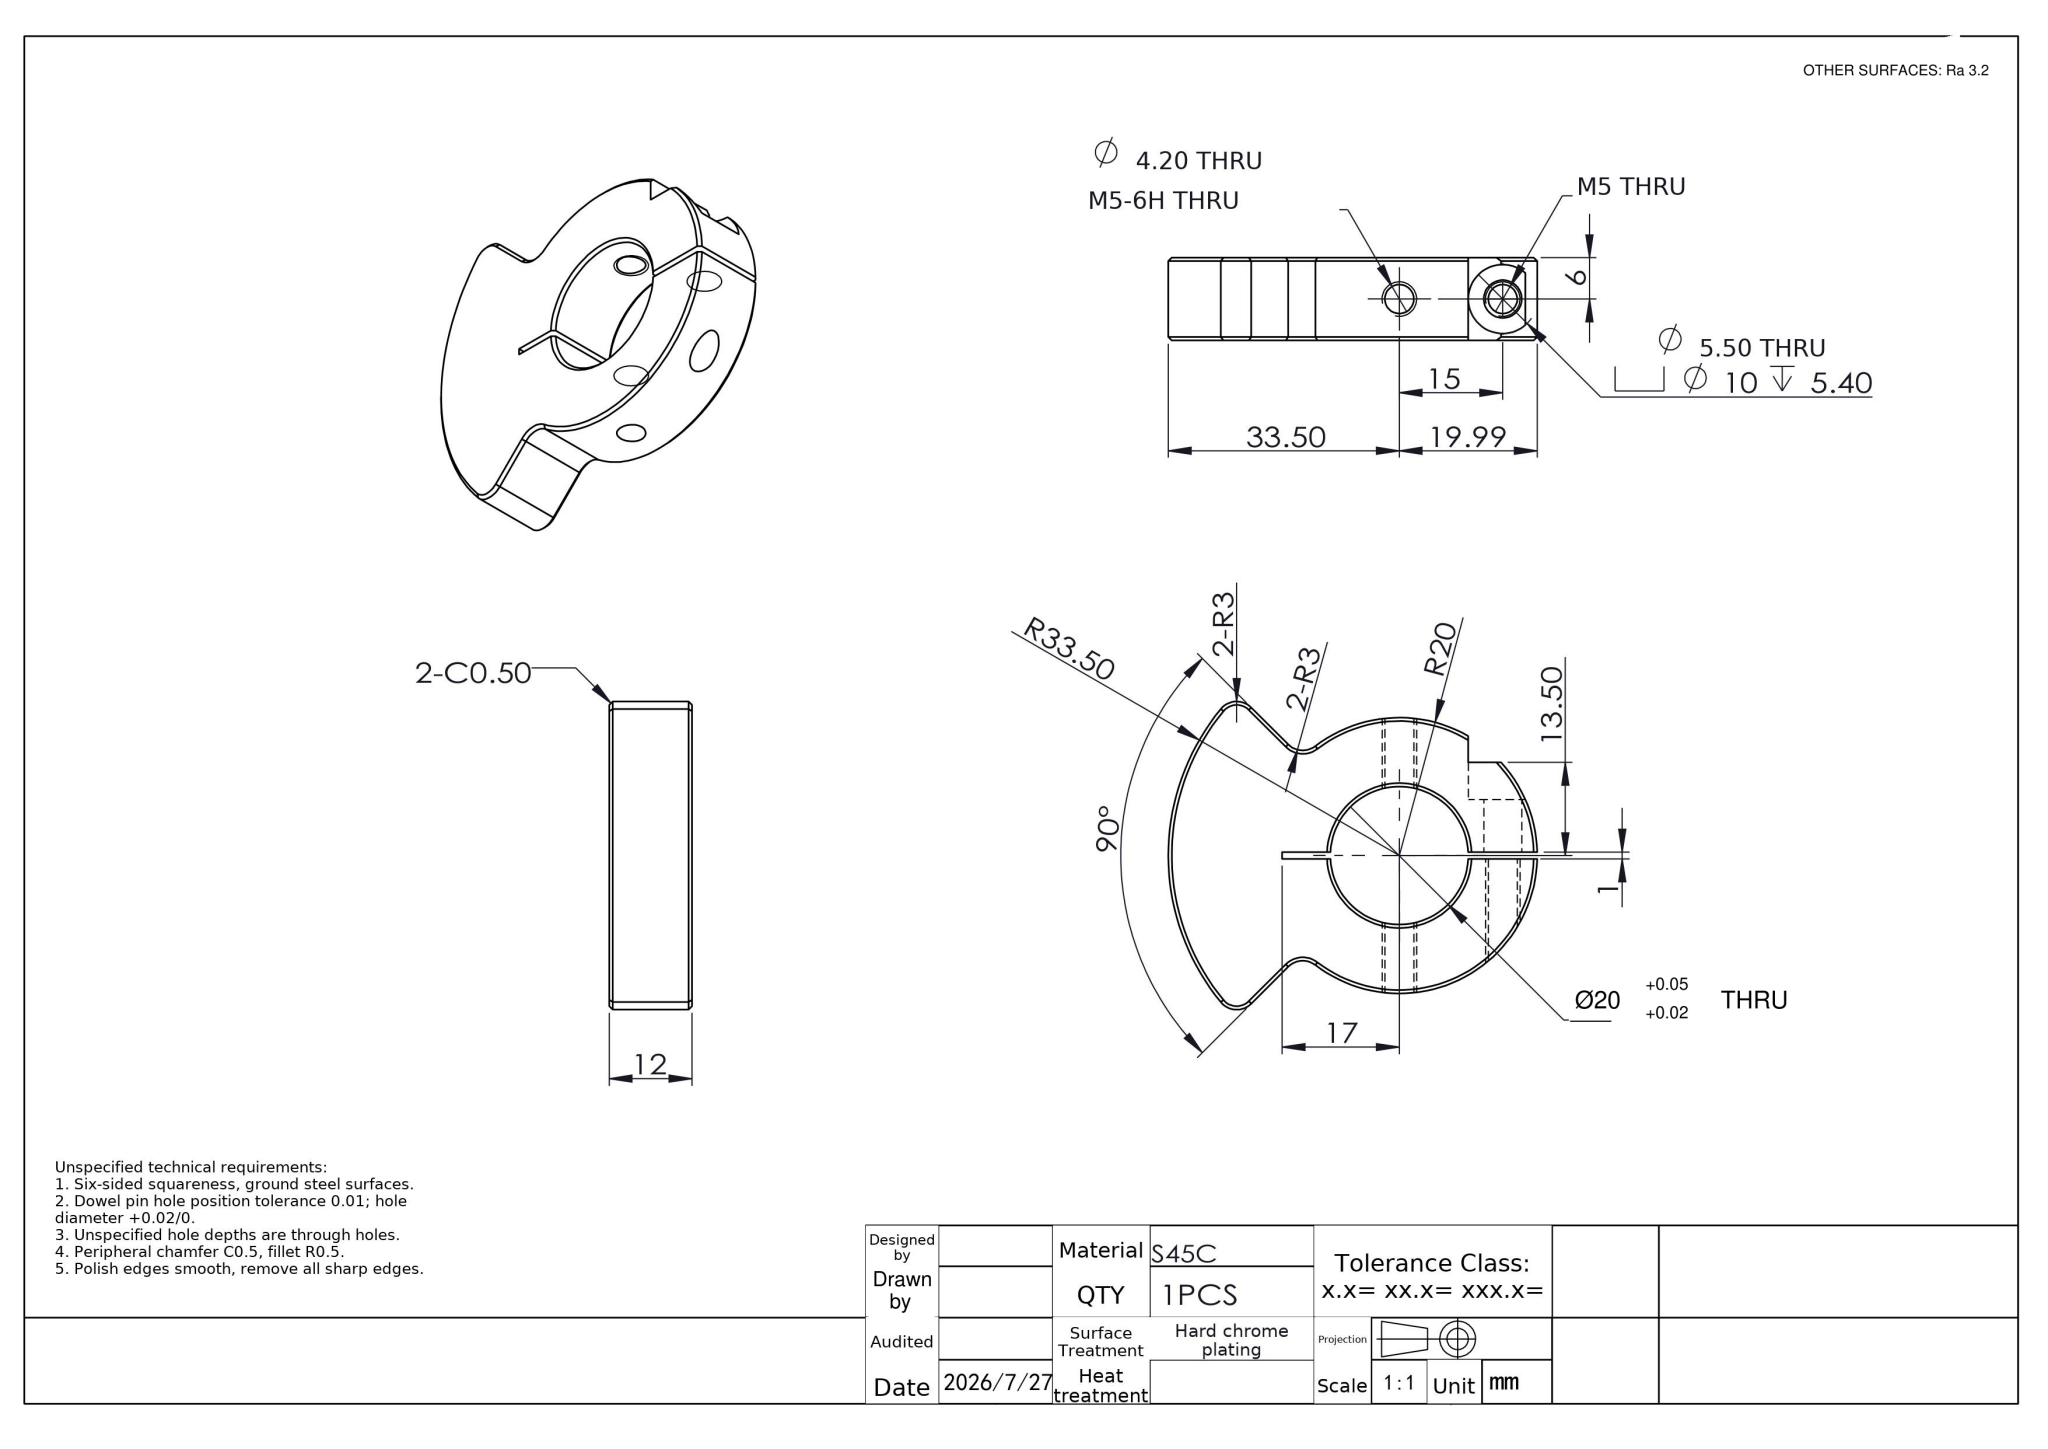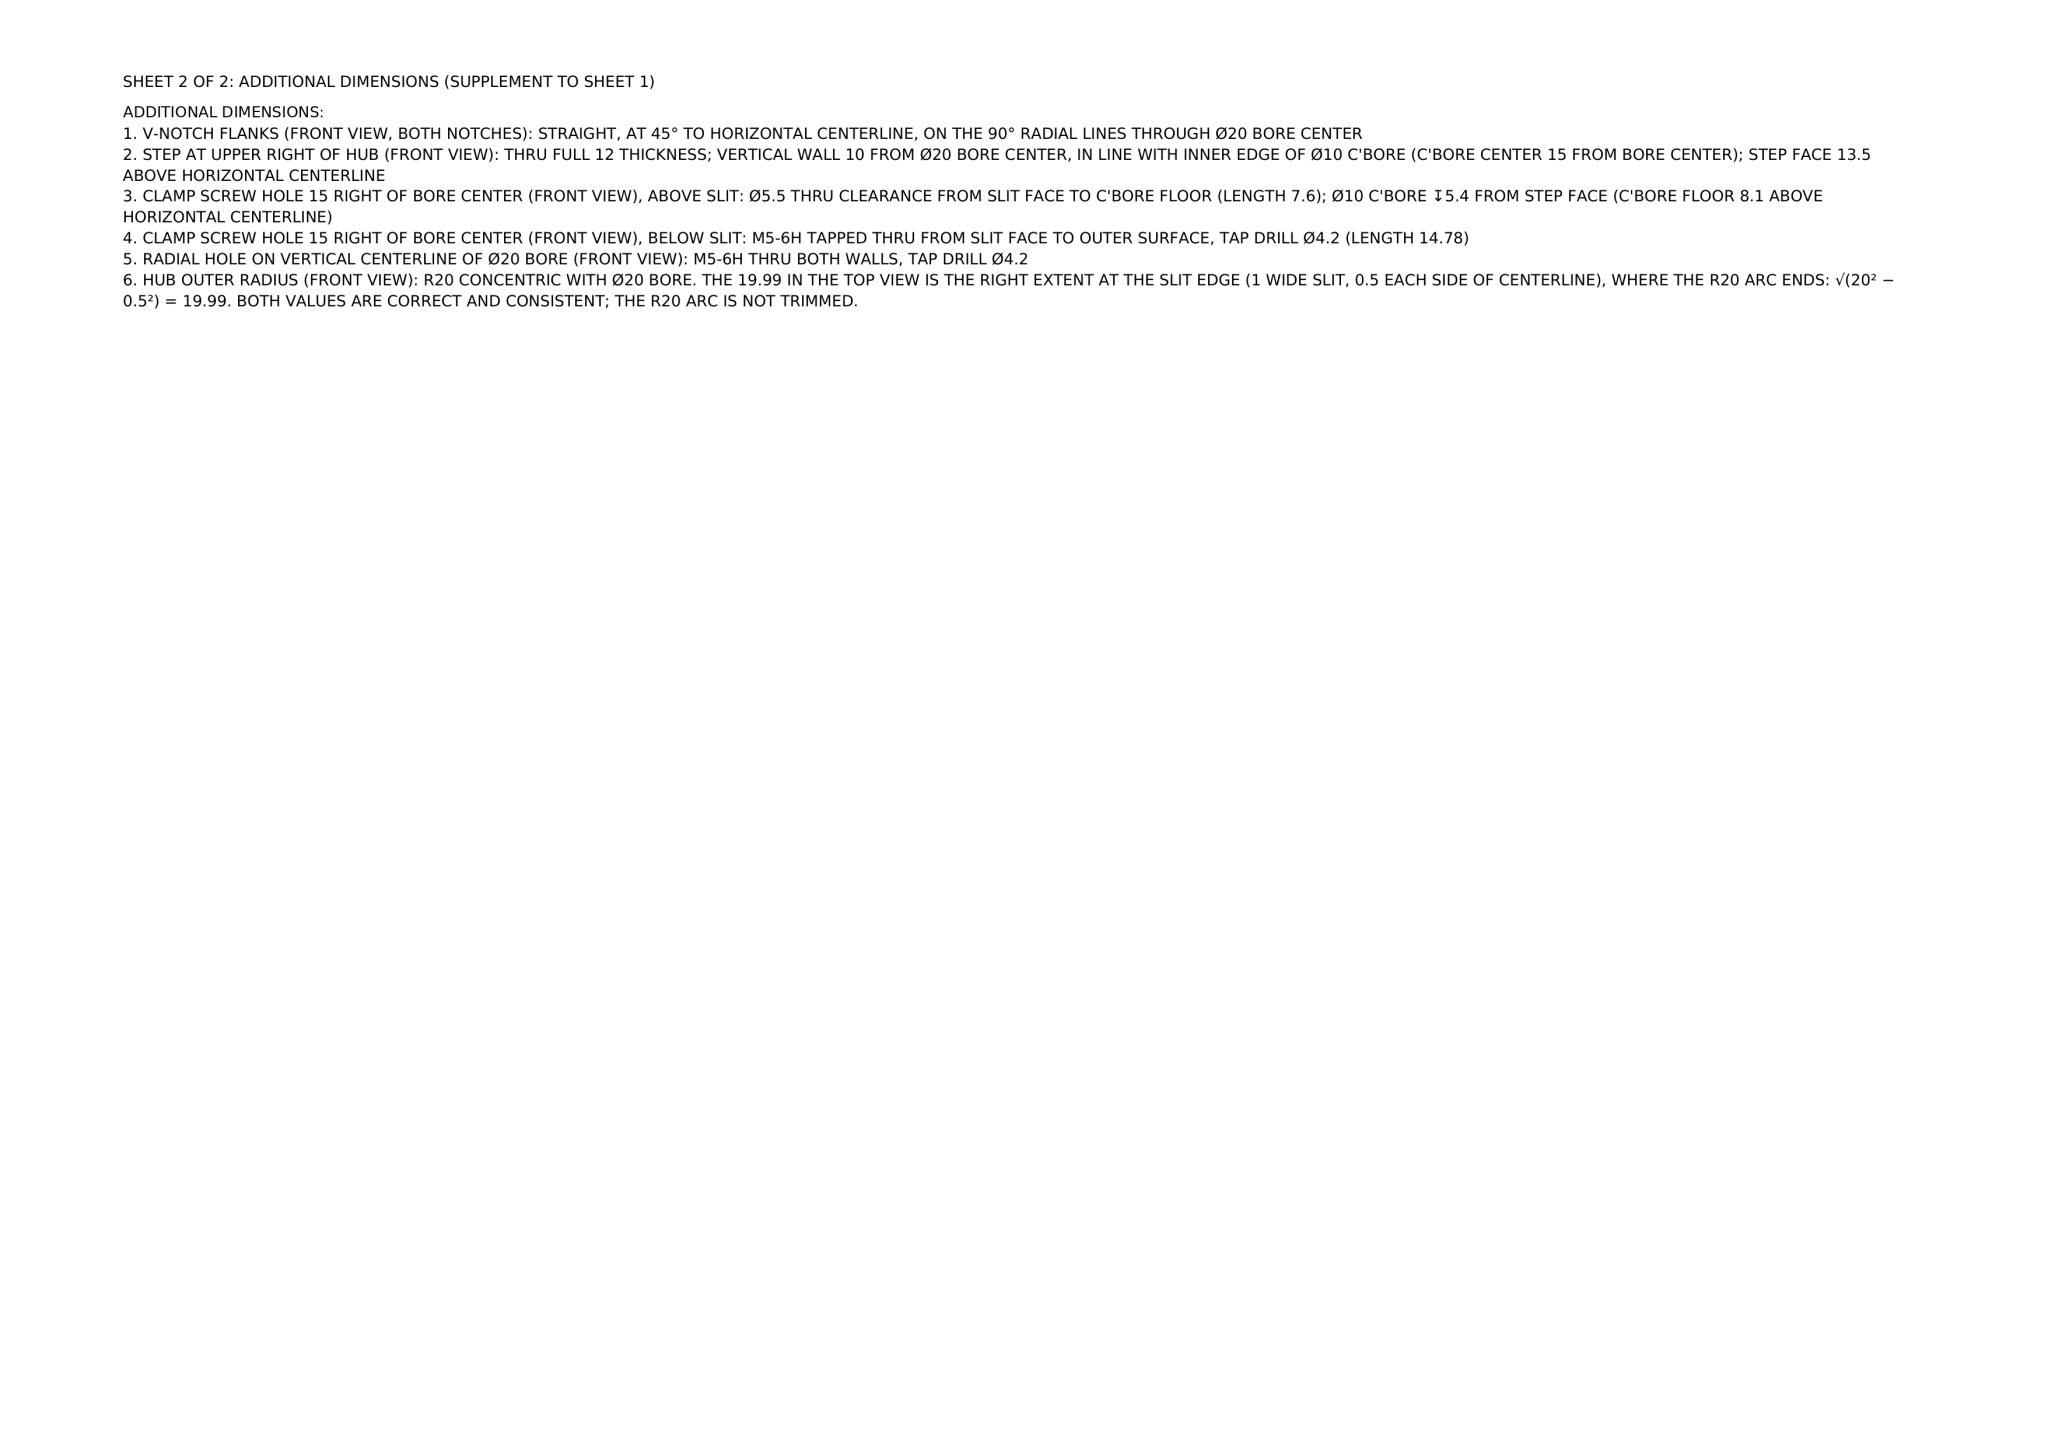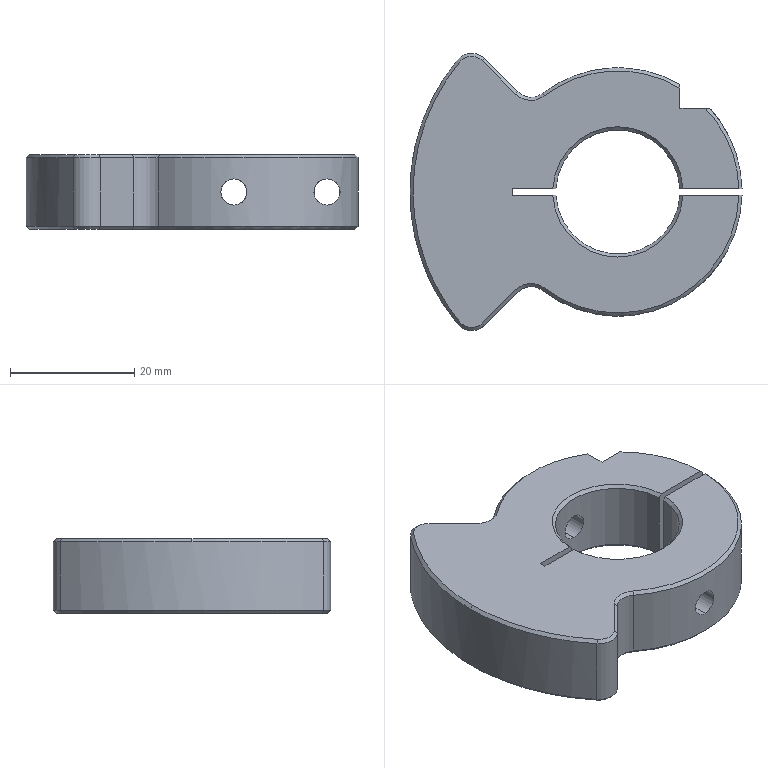Part | NX | mm | 1 solid | 59 faces | box 53.49 x 44.68 x 12 mm | volume 16785 mm3 | cylinder 21 | cone 21 | plane 17 | commonest cylinder face diameters 4.2 x6 6 x4 10 x3 40 x3 5.5 x2 20 x2 67 x1